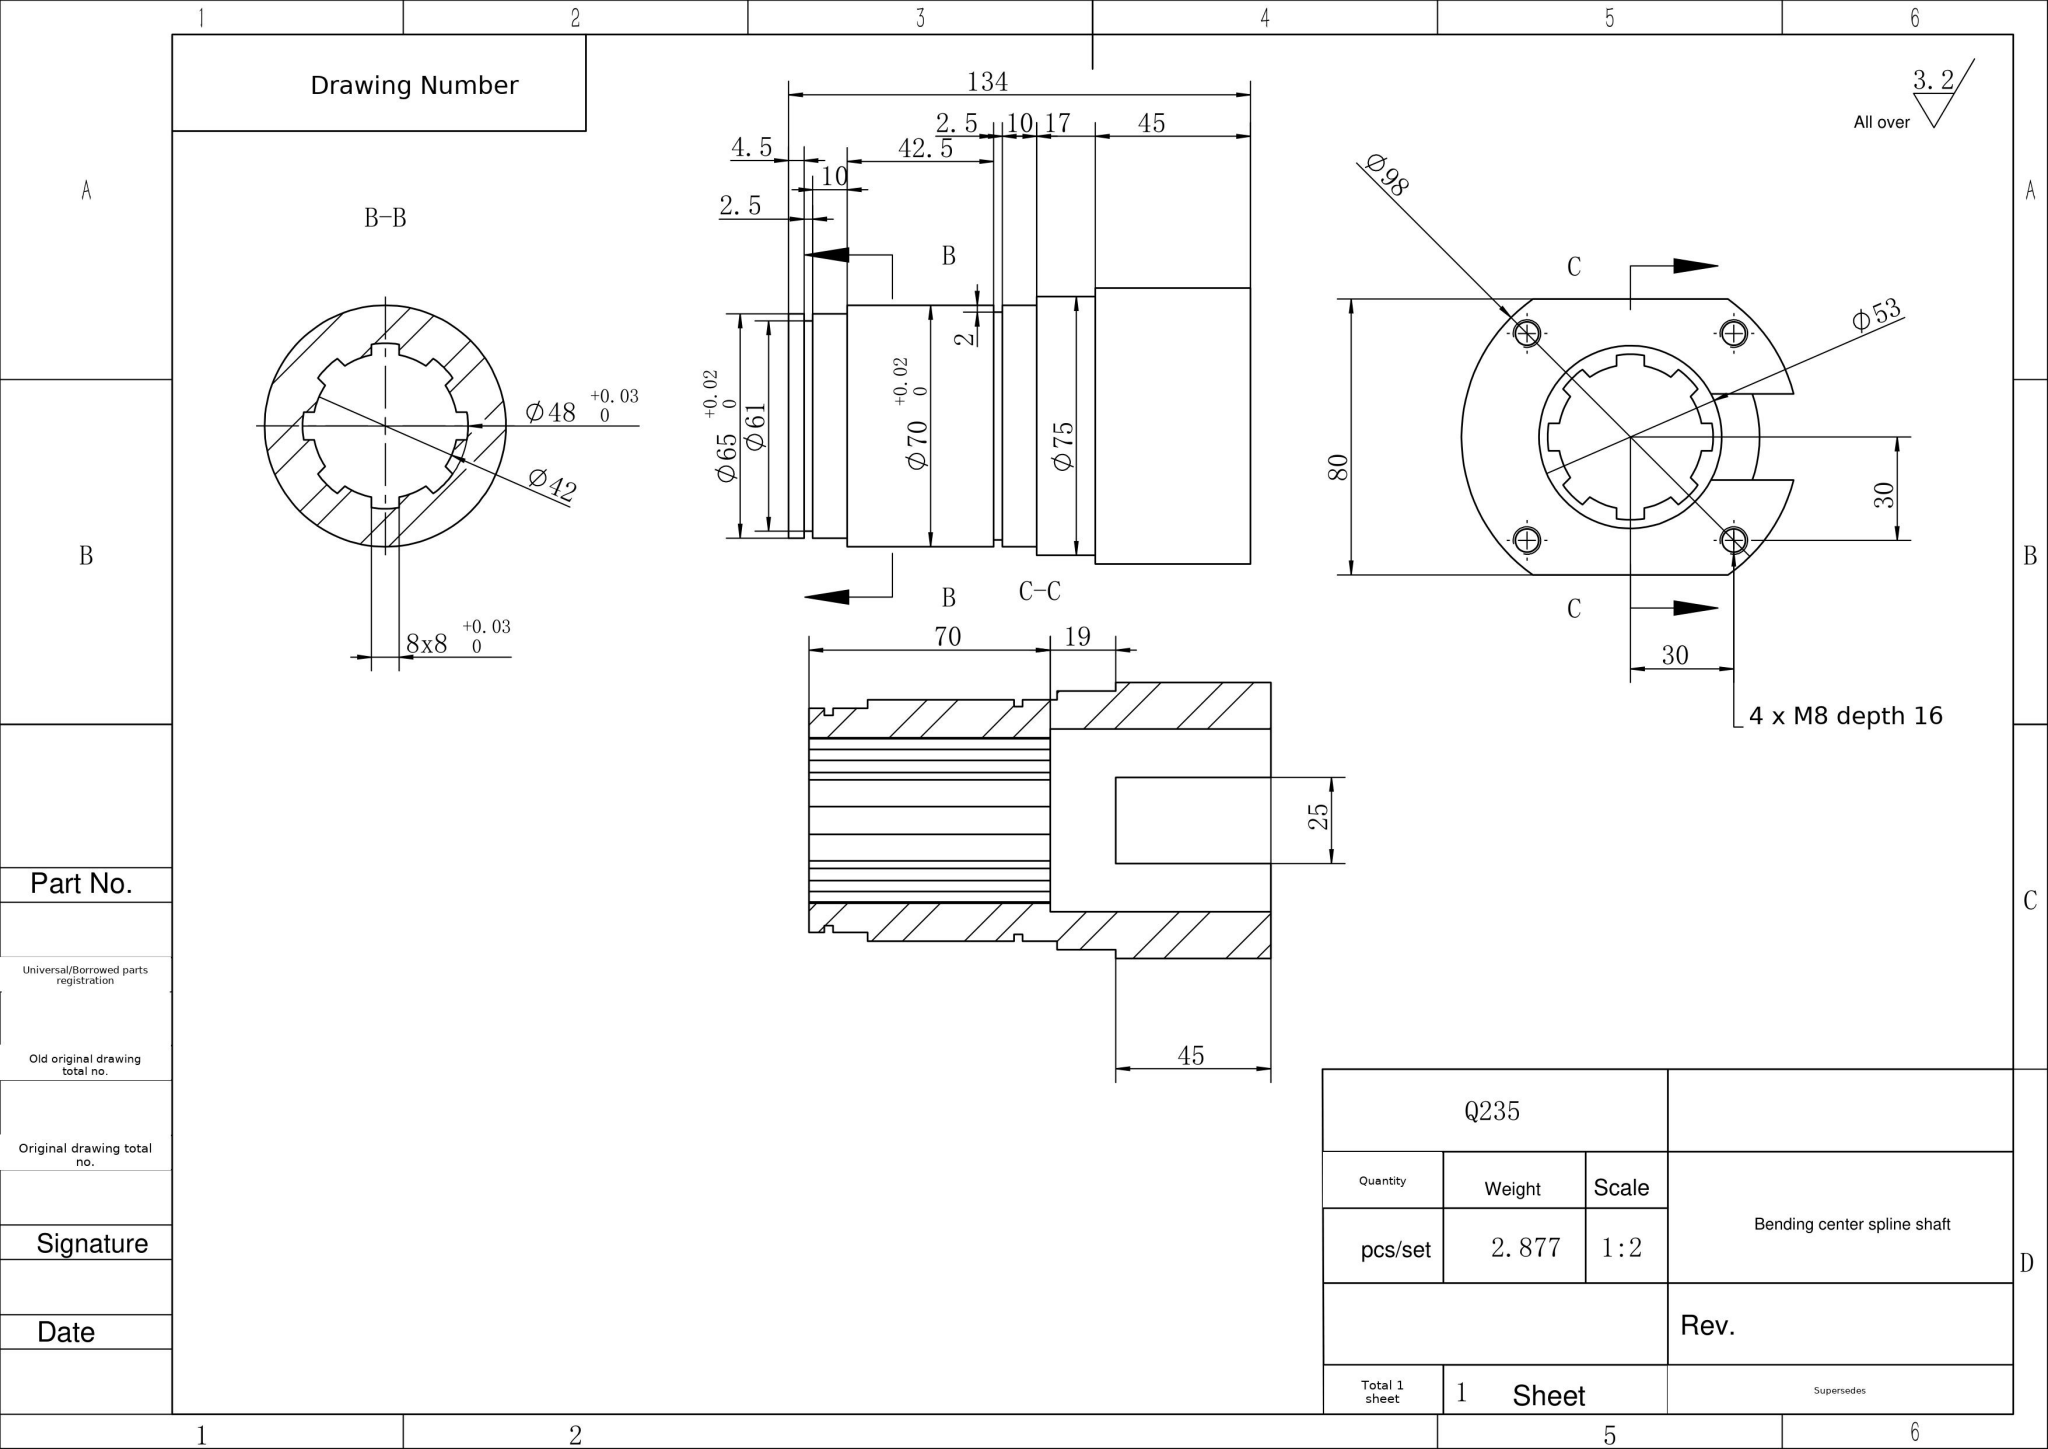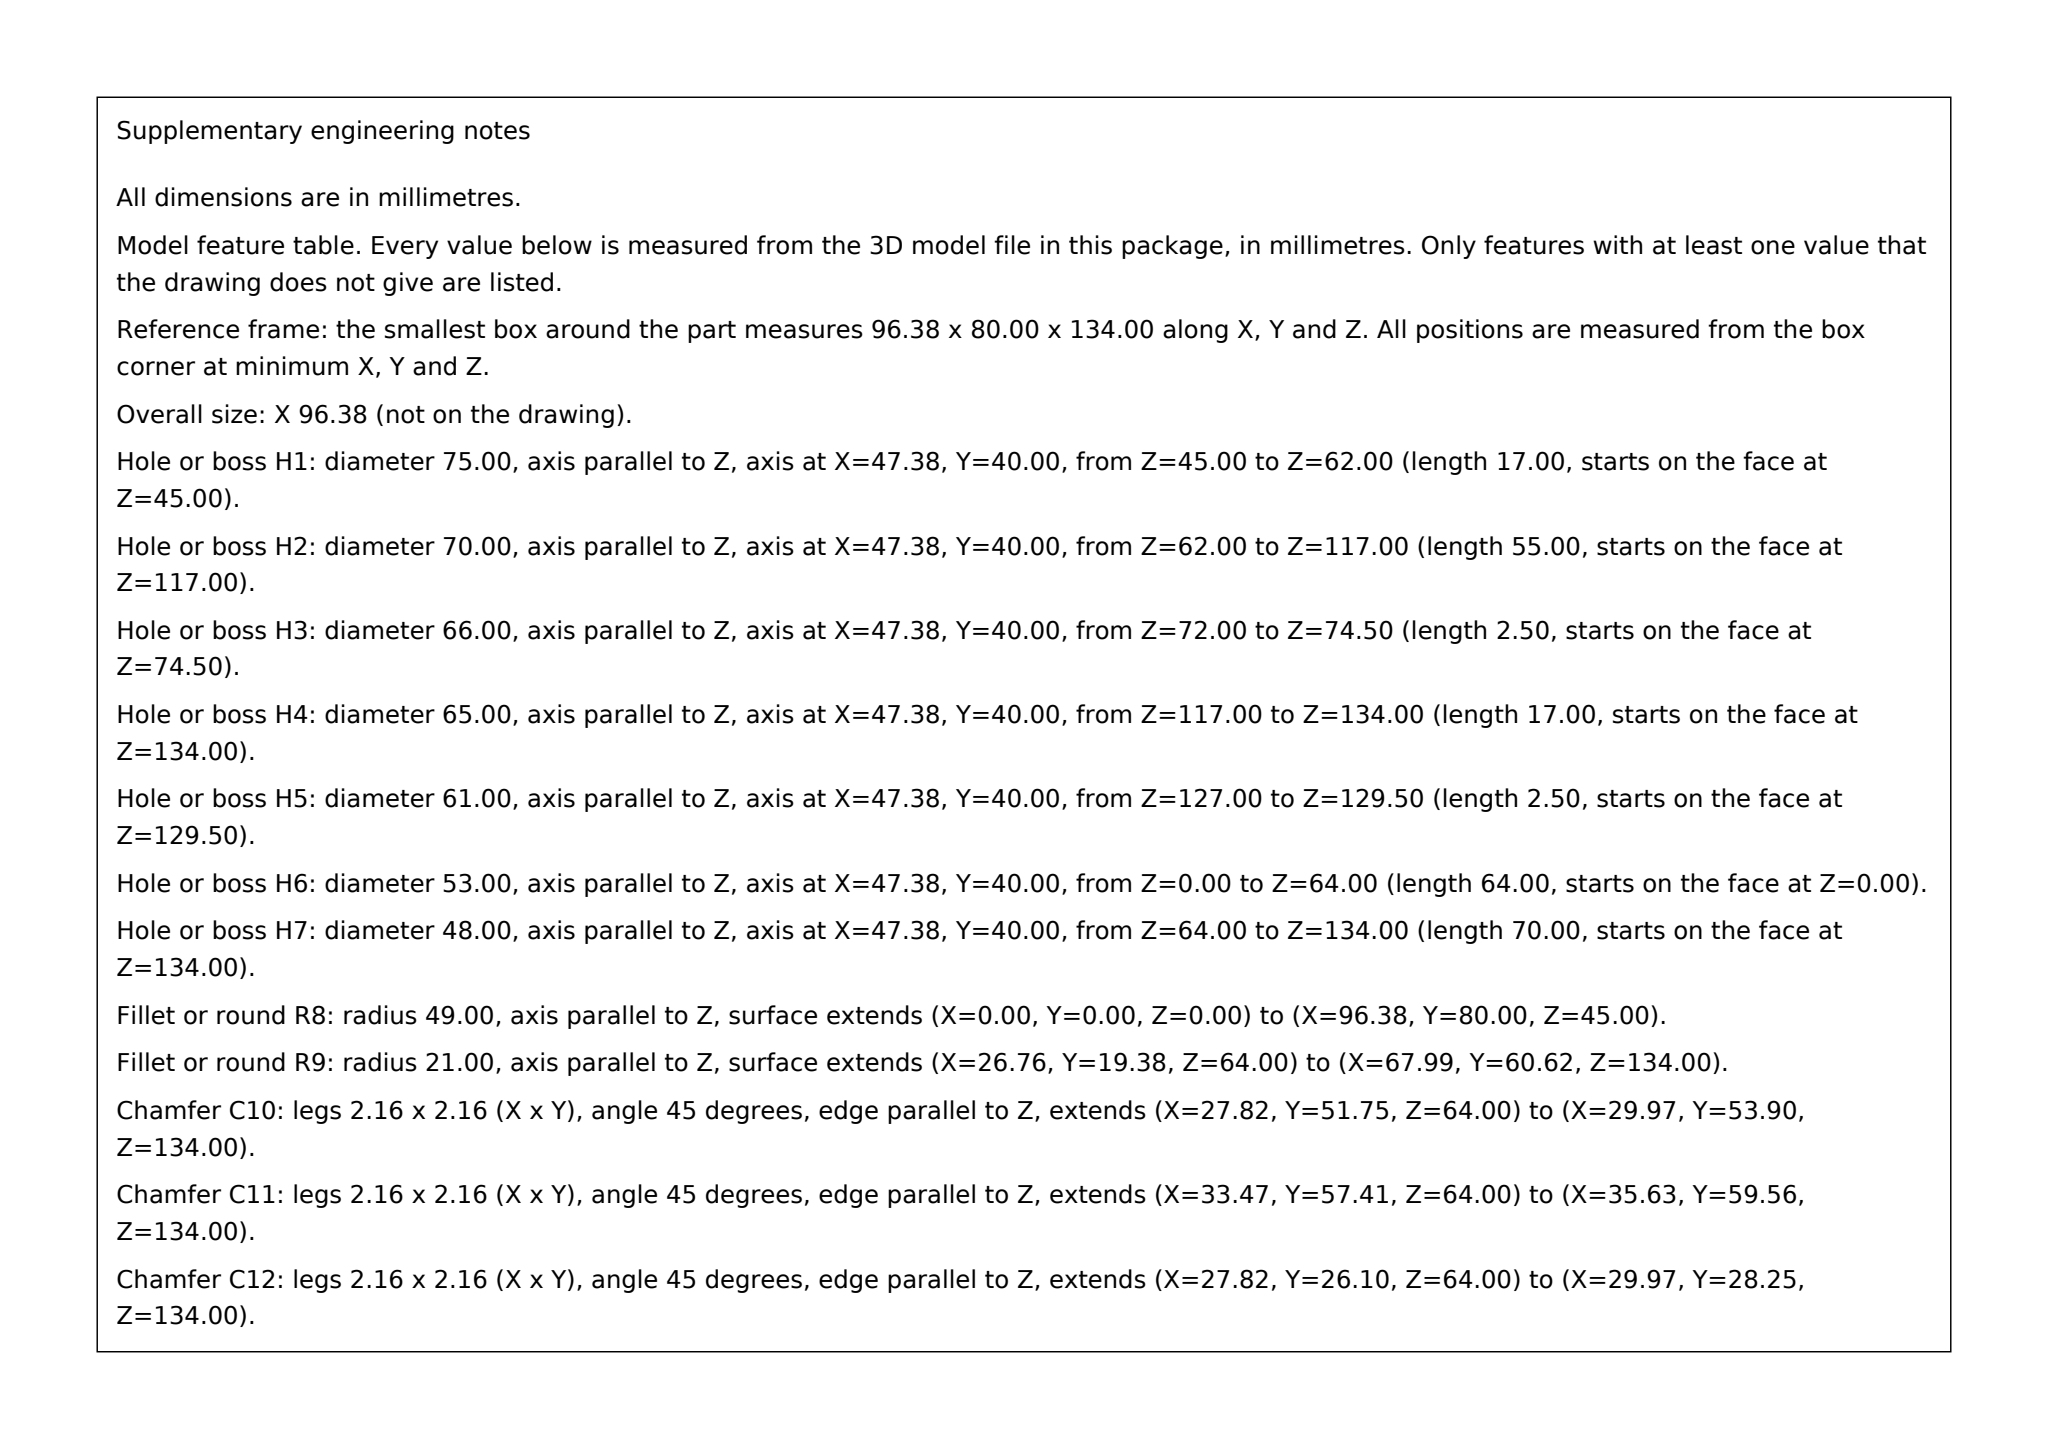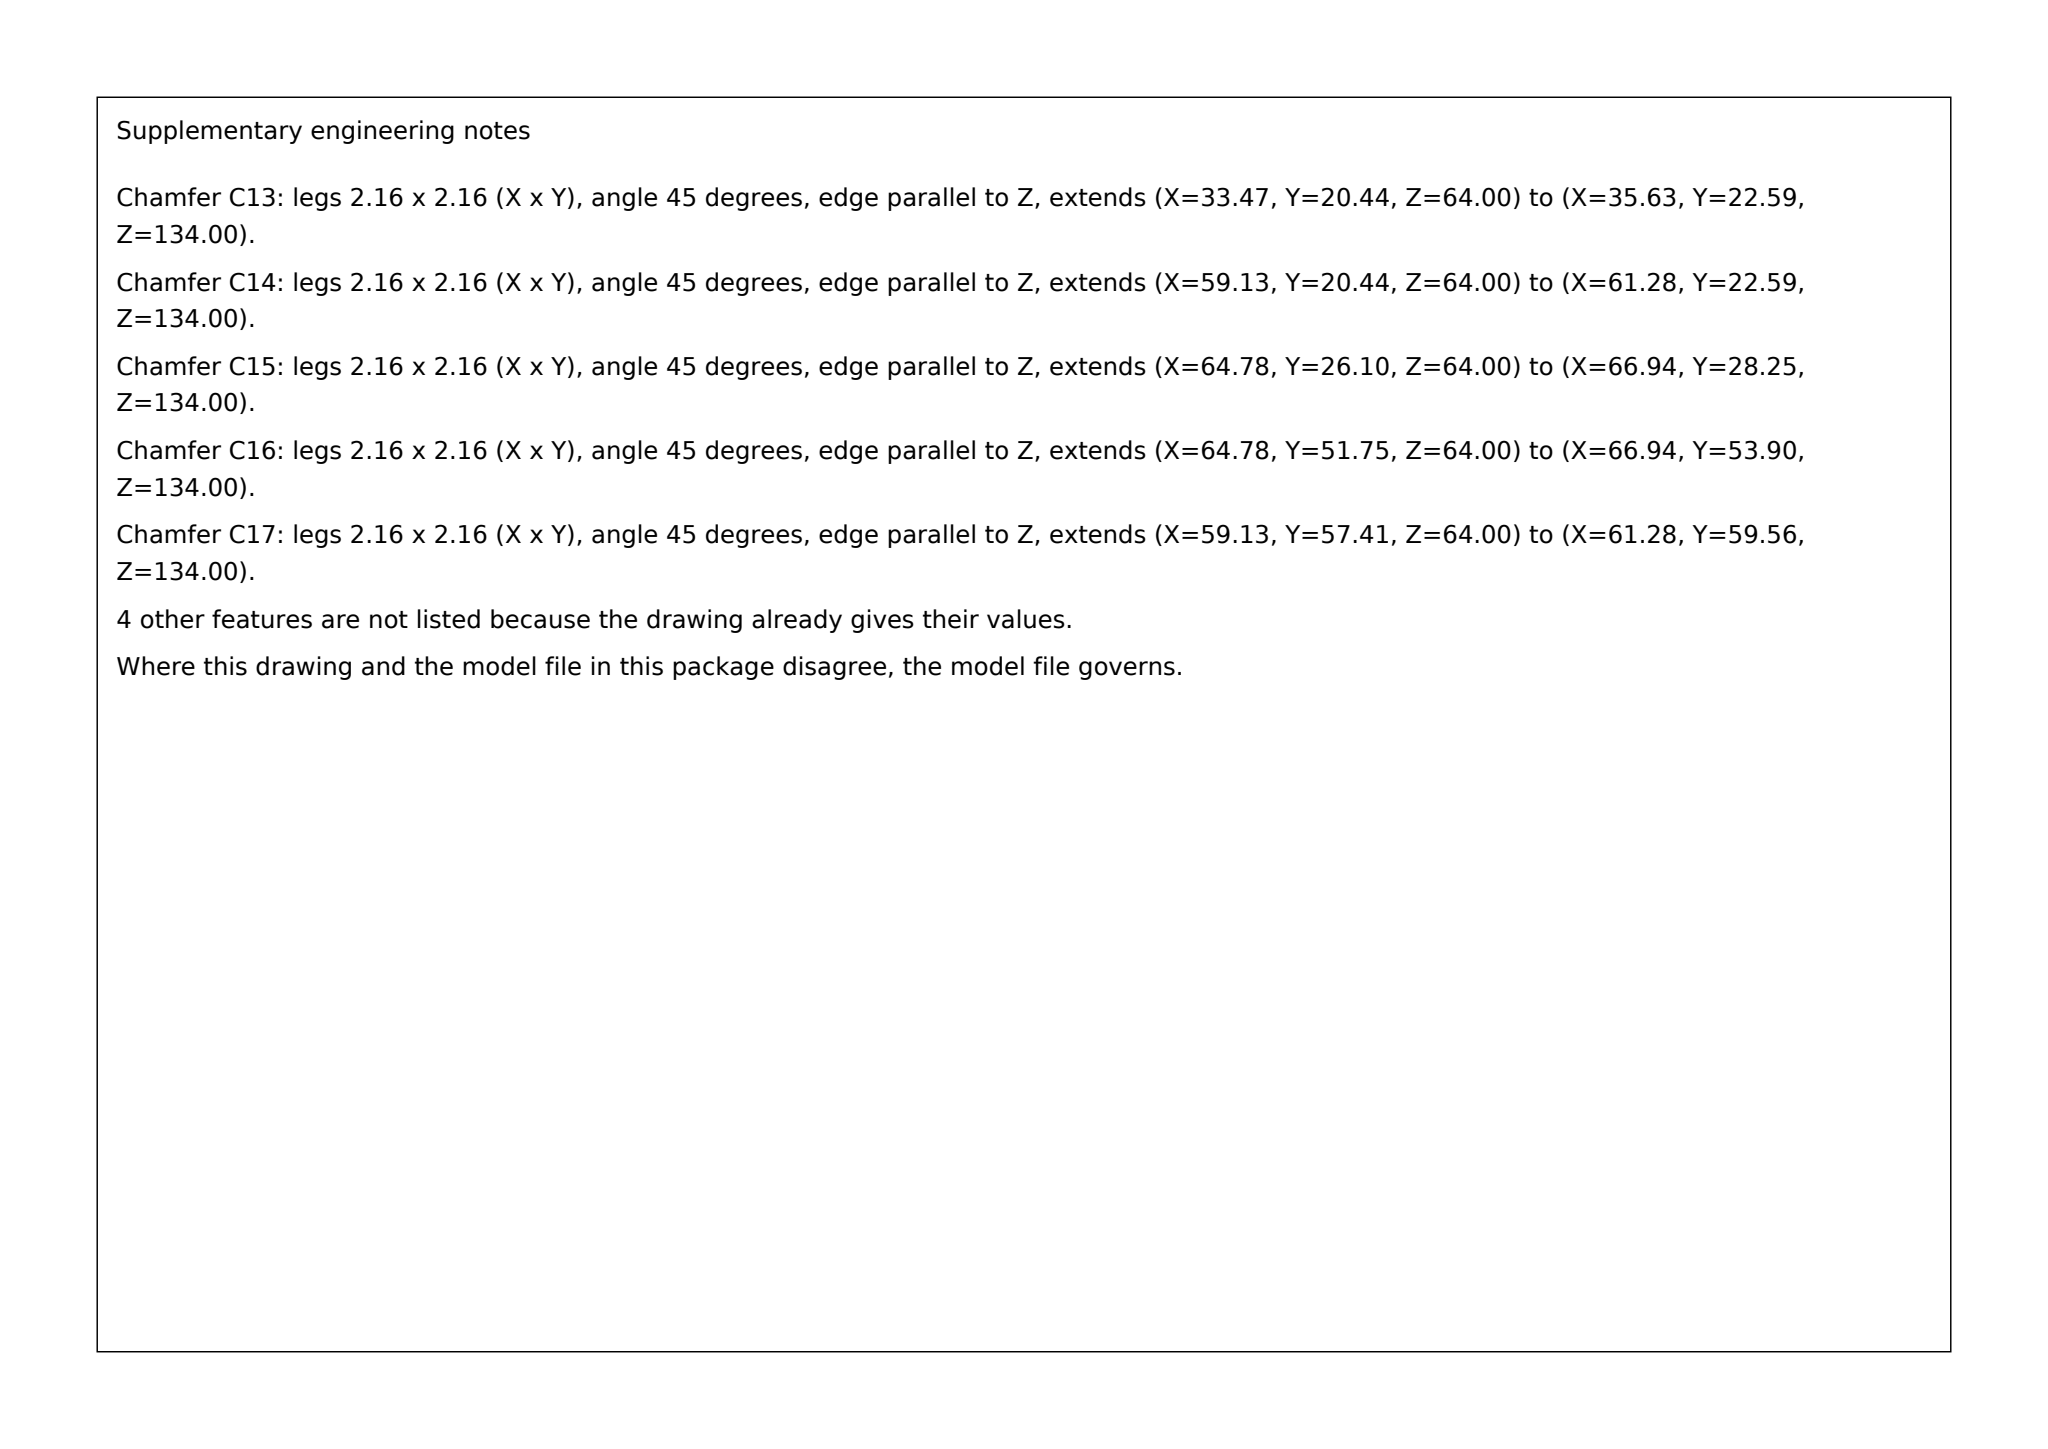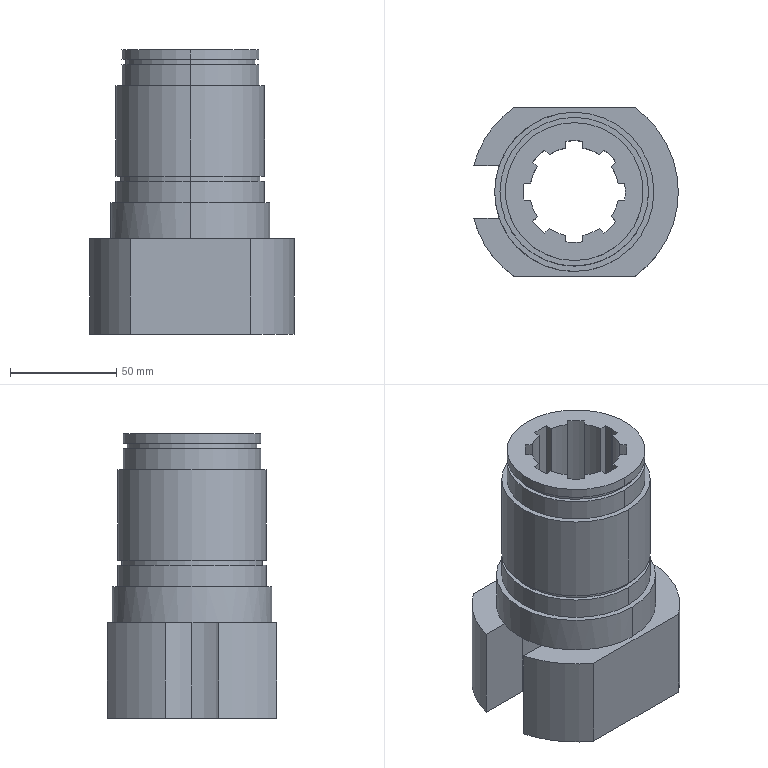Part | SolidWorks | mm | material Q235 | 1 solid | 83 faces | box 96.38 x 80 x 134 mm | volume 368869 mm3 | cylinder 44 | plane 31 | cone 8 | commonest cylinder face diameters 48 x9 6.8 x8 42 x8 65 x4 70 x4 98 x3 53 x2 61 x2
build123d program:
from build123d import *

# Parameters (mm, degrees)
BOSS_EXTRUDE1_DEPTH   = 20
BOSS_EXTRUDE2_DEPTH   = 25
SKETCH5_R             = 22.5
CUT_EXTRUDE1_DEPTH    = 10
CUT_EXTRUDE2_DEPTH    = 45
SKETCH8_R             = 26.5
CUT_EXTRUDE3_DEPTH    = 48
CUT_EXTRUDE4_START    = -70
CUT_EXTRUDE4_DEPTH    = 70
M8_TAPPED_HOLE1_D     = 6.8
M8_TAPPED_HOLE1_DEPTH = 19.75
M8_TAPPED_HOLE1_TIP   = 2.043
CUT_EXTRUDE9_START    = -16
SKETCH23_R            = 26.5
CUT_EXTRUDE9_DEPTH    = 16


with BuildPart() as part:
    # Sketch1 → Boss-Extrude1 (new body)
    with BuildSketch(Plane.XY):
        with BuildLine():
            Line((-28.302, 40), (28.302, 40))
            ThreePointArc((28.302, 40), (49, 0), (28.302, -40))
            Line((28.302, -40), (-28.302, -40))
            ThreePointArc((-28.302, -40), (-49, 0), (-28.302, 40))
        make_face()
    extrude(amount=BOSS_EXTRUDE1_DEPTH)

    # Sketch3 → Boss-Extrude2 (add)
    with BuildSketch(Plane.XY.offset(20)):
        with BuildLine():
            Line((-28.302, 40), (28.302, 40))
            ThreePointArc((28.302, 40), (49, 0), (28.302, -40))
            Line((28.302, -40), (-28.302, -40))
            ThreePointArc((-28.302, -40), (-49, 0), (-28.302, 40))
        make_face()
    extrude(amount=BOSS_EXTRUDE2_DEPTH)

    # Sketch4 → Revolve1 (revolve)
    with BuildSketch(Plane(origin=(0, 0, 0), x_dir=(0, 0, -1), z_dir=(1, 0, 0)), mode=Mode.PRIVATE) as revolve1_sk:
        Polygon((-45, 0), (-45, 37.5), (-62, 37.5), (-62, 35), (-72, 35), (-72, 33), (-74.5, 33), (-74.5, 35), (-117, 35), (-117, 32.5), (-127, 32.5), (-127, 30.5), (-129.5, 30.5), (-129.5, 32.5), (-134, 32.5), (-134, 21), (-64, 21), (-64, 0), align=None)
    revolve(revolve1_sk.sketch.rotate(Axis((0, 0, 64), (0, 0, -1)), 180), axis=Axis((0, 0, 64), (0, 0, -1)))

    # Sketch5 → Cut-Extrude1 (cut)
    with BuildSketch(Plane(origin=(0, 0, 0), x_dir=(-1, 0, 0), z_dir=(0, 0, -1))):
        Circle(SKETCH5_R)
    extrude(amount=-CUT_EXTRUDE1_DEPTH, mode=Mode.SUBTRACT)

    # Sketch7 → Cut-Extrude2 (cut)
    with BuildSketch(Plane(origin=(0, 0, 0), x_dir=(-1, 0, 0), z_dir=(0, 0, -1))):
        with BuildLine():
            Line((0, 12.5), (82.765, 12.5))
            Line((82.765, 12.5), (82.765, -12.5))
            Line((82.765, -12.5), (0, -12.5))
            ThreePointArc((0, -12.5), (-12.5, 0), (0, 12.5))
        make_face()
    extrude(amount=-CUT_EXTRUDE2_DEPTH, mode=Mode.SUBTRACT)

    # Sketch8 → Cut-Extrude3 (cut)
    with BuildSketch(Plane.XY.offset(64)):
        Circle(SKETCH8_R)
    extrude(amount=-CUT_EXTRUDE3_DEPTH, mode=Mode.SUBTRACT)

    # Sketch10 → Cut-Extrude4 (cut)
    with BuildSketch(Plane.XY.offset(134).offset(CUT_EXTRUDE4_START)):
        with BuildLine():
            Line((13.905, 19.562), (11.749, 17.406))
            ThreePointArc((11.749, 17.406), (8.036, 19.401), (4, 20.616))
            Line((4, 20.616), (4, 23.664))
            ThreePointArc((4, 23.664), (0, 24), (-4, 23.664))
            Line((-4, 23.664), (-4, 20.616))
            ThreePointArc((-4, 20.616), (-8.036, 19.401), (-11.749, 17.406))
            Line((-11.749, 17.406), (-13.905, 19.562))
            ThreePointArc((-13.905, 19.562), (-16.971, 16.971), (-19.562, 13.905))
            Line((-19.562, 13.905), (-17.406, 11.749))
            ThreePointArc((-17.406, 11.749), (-19.401, 8.036), (-20.616, 4))
            Line((-20.616, 4), (-23.664, 4))
            ThreePointArc((-23.664, 4), (-24, 0), (-23.664, -4))
            Line((-23.664, -4), (-20.616, -4))
            ThreePointArc((-20.616, -4), (-19.401, -8.036), (-17.406, -11.749))
            Line((-17.406, -11.749), (-19.562, -13.905))
            ThreePointArc((-19.562, -13.905), (-16.971, -16.971), (-13.905, -19.562))
            Line((-13.905, -19.562), (-11.749, -17.406))
            ThreePointArc((-11.749, -17.406), (-8.036, -19.401), (-4, -20.616))
            Line((-4, -20.616), (-4, -23.664))
            ThreePointArc((-4, -23.664), (0, -24), (4, -23.664))
            Line((4, -23.664), (4, -20.616))
            ThreePointArc((4, -20.616), (8.036, -19.401), (11.749, -17.406))
            Line((11.749, -17.406), (13.905, -19.562))
            ThreePointArc((13.905, -19.562), (16.971, -16.971), (19.562, -13.905))
            Line((19.562, -13.905), (17.406, -11.749))
            ThreePointArc((17.406, -11.749), (19.401, -8.036), (20.616, -4))
            Line((20.616, -4), (23.664, -4))
            ThreePointArc((23.664, -4), (24, 0), (23.664, 4))
            Line((23.664, 4), (20.616, 4))
            ThreePointArc((20.616, 4), (19.401, 8.036), (17.406, 11.749))
            Line((17.406, 11.749), (19.562, 13.905))
            ThreePointArc((19.562, 13.905), (16.971, 16.971), (13.905, 19.562))
        make_face()
    extrude(amount=CUT_EXTRUDE4_DEPTH, mode=Mode.SUBTRACT)

    # M8 Tapped Hole1
    with Locations(Plane(origin=(30, 30, 0), x_dir=(-1, 0, 0), z_dir=(0, 0, -1))):
        with Locations((0, 0), (60, 0), (60, -60), (0, -60)):
            Hole(M8_TAPPED_HOLE1_D / 2, depth=M8_TAPPED_HOLE1_DEPTH)
            with Locations((0, 0, -(M8_TAPPED_HOLE1_DEPTH + M8_TAPPED_HOLE1_TIP / 2))):  # 118° drill point
                Cone(0, M8_TAPPED_HOLE1_D / 2, M8_TAPPED_HOLE1_TIP, mode=Mode.SUBTRACT)

    # Sketch23 → Cut-Extrude9 (cut)
    with BuildSketch(Plane(origin=(0, 0, 0), x_dir=(-1, 0, 0), z_dir=(0, 0, -1)).offset(CUT_EXTRUDE9_START)):
        with Locations(Location((0, 0, 0), (0, 0, 180))):
            Circle(SKETCH23_R)
    extrude(amount=CUT_EXTRUDE9_DEPTH, mode=Mode.SUBTRACT)


solid = part.part